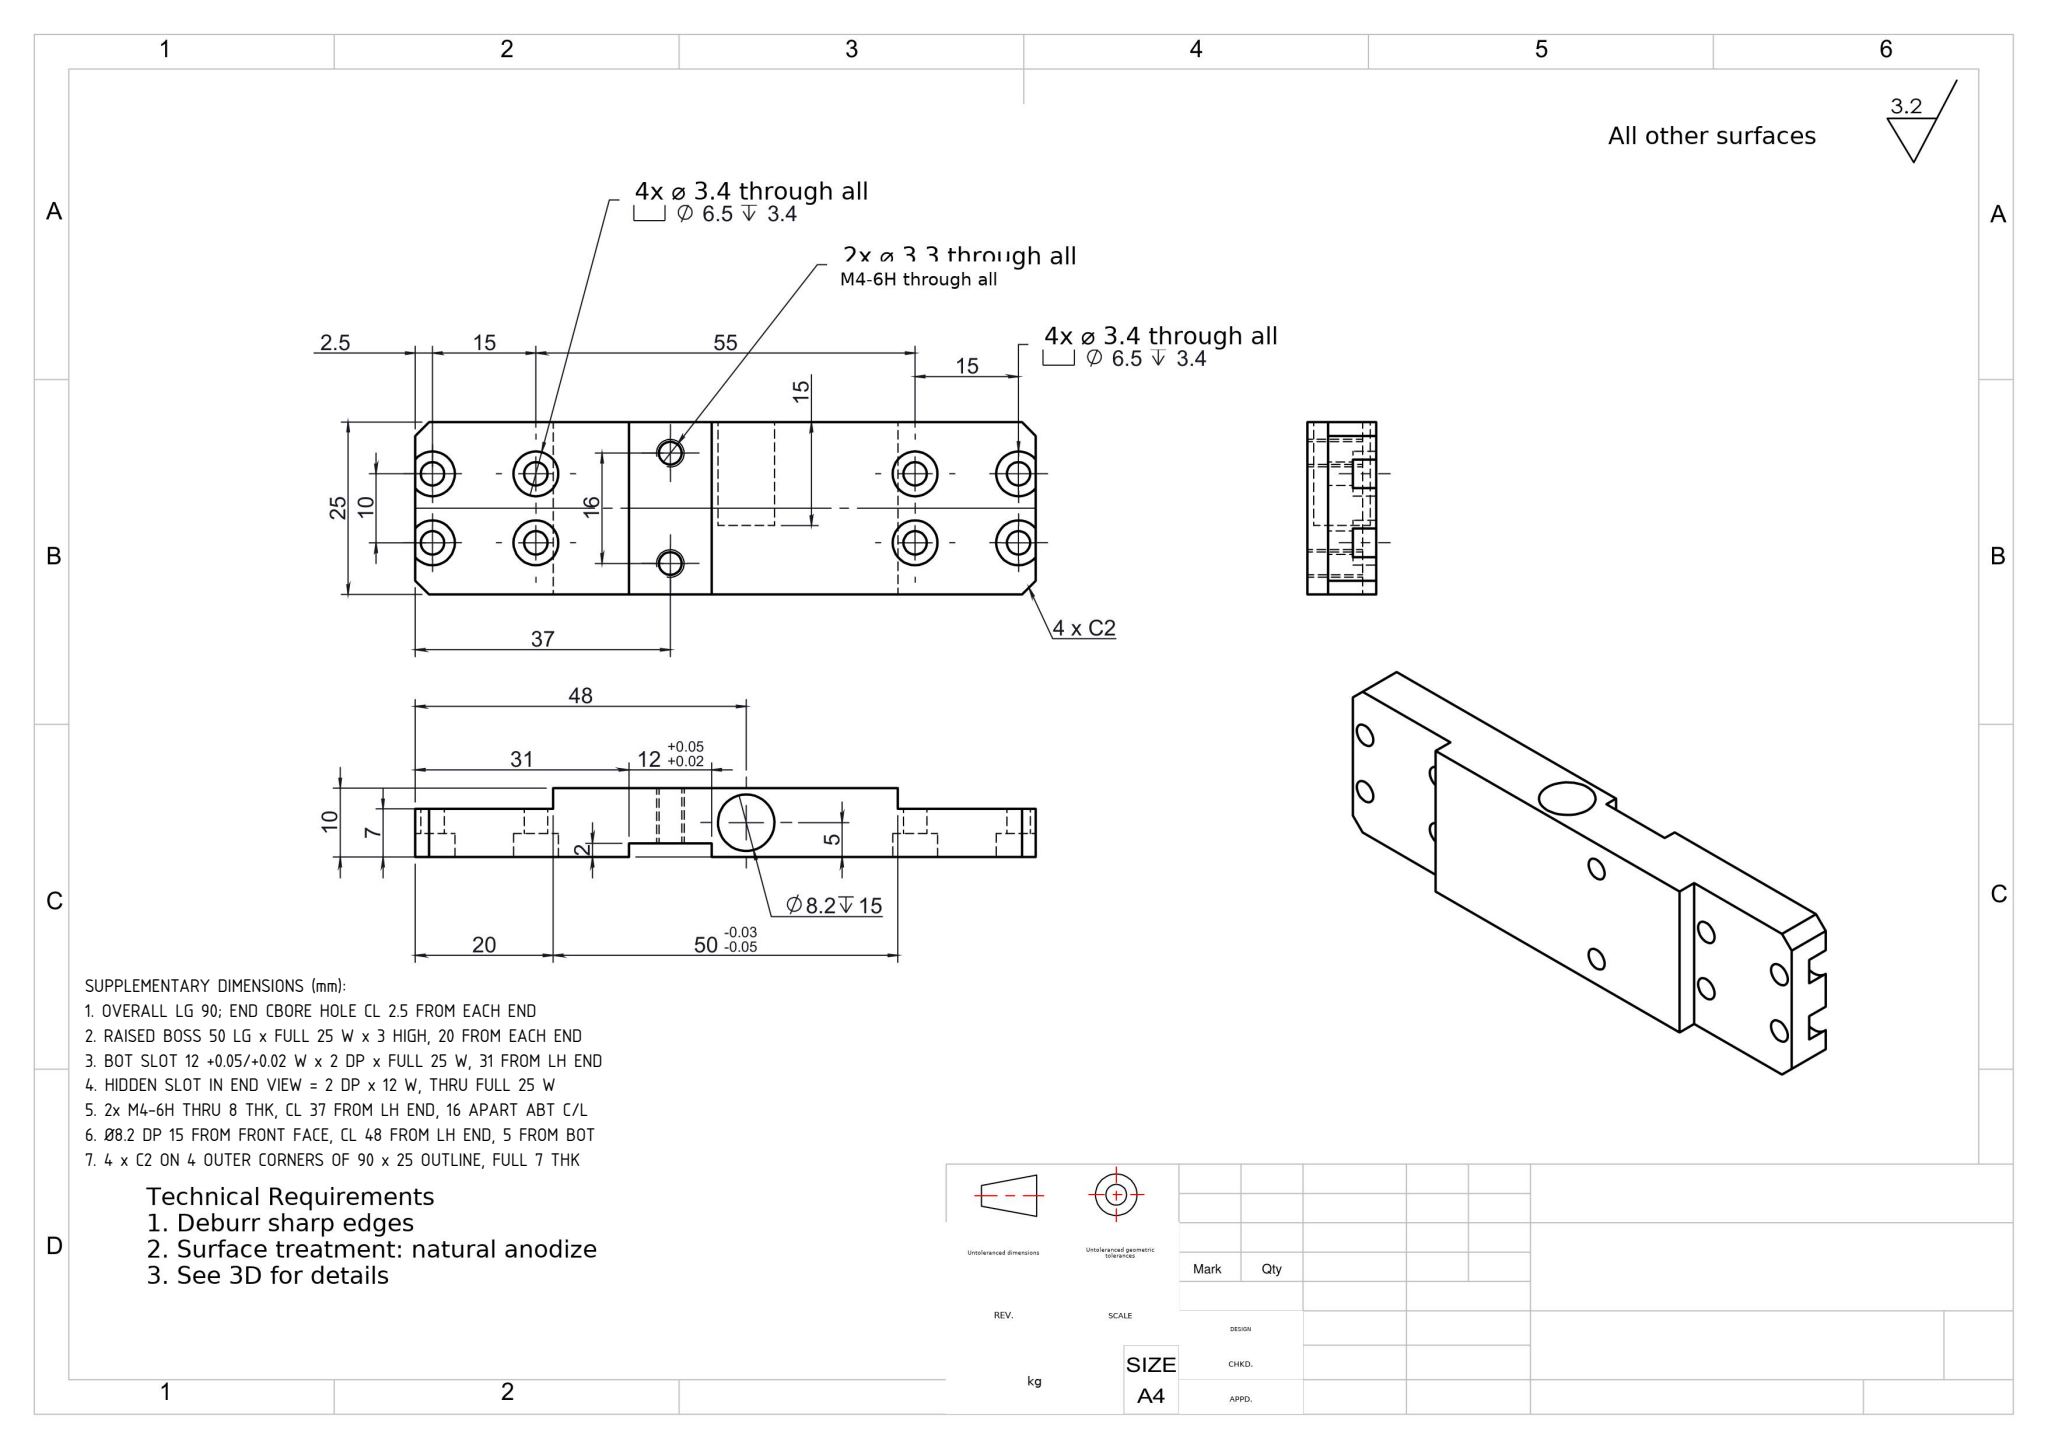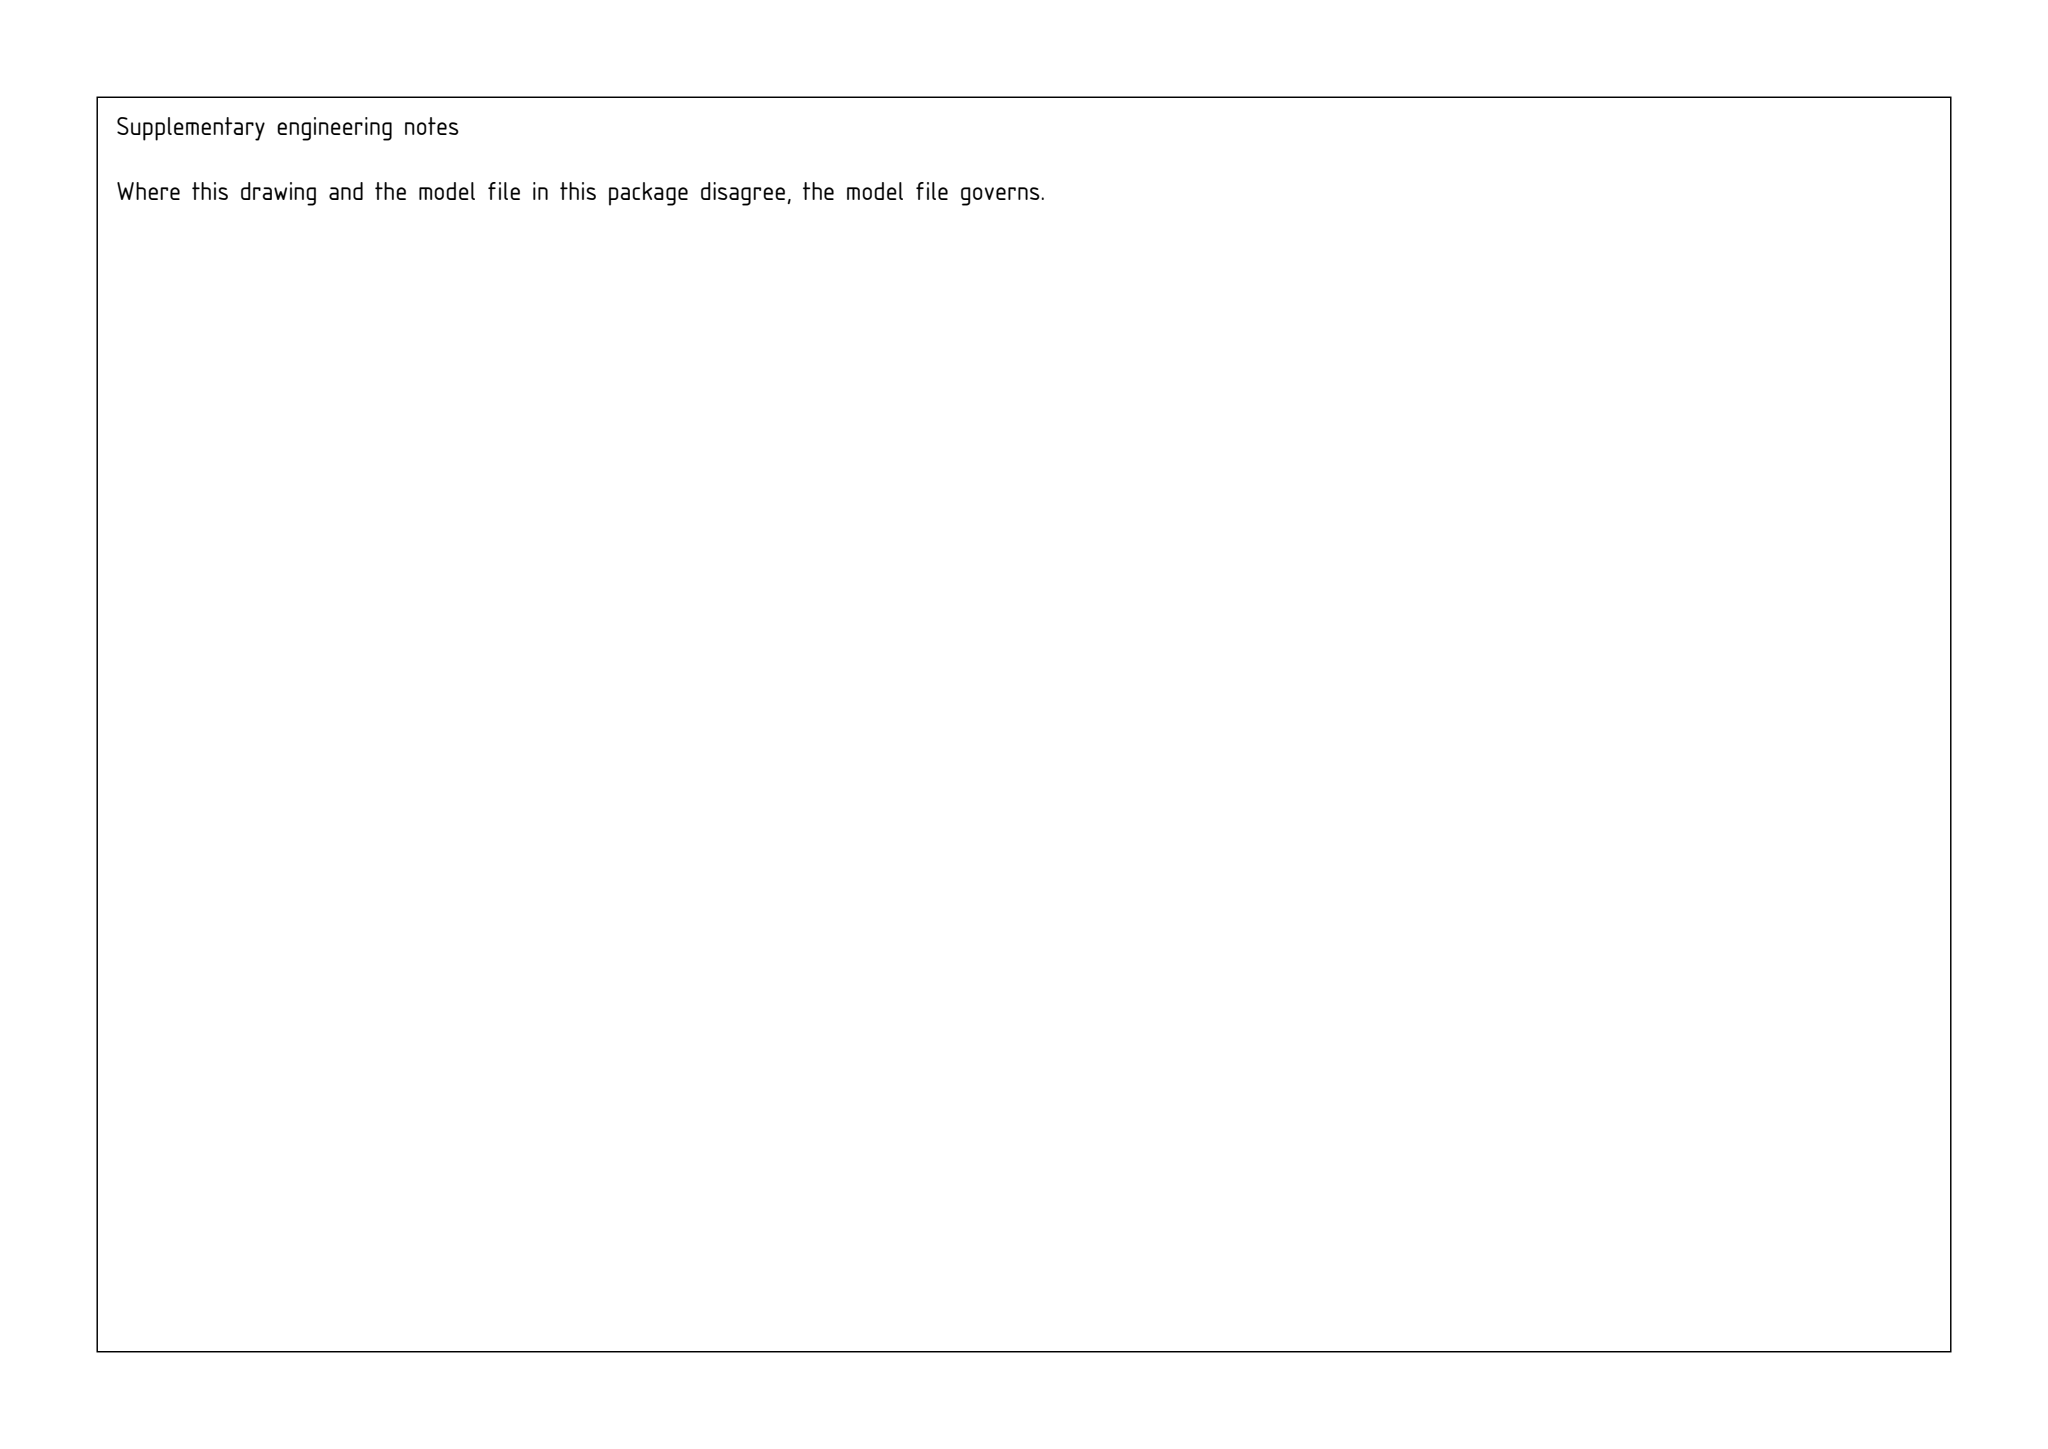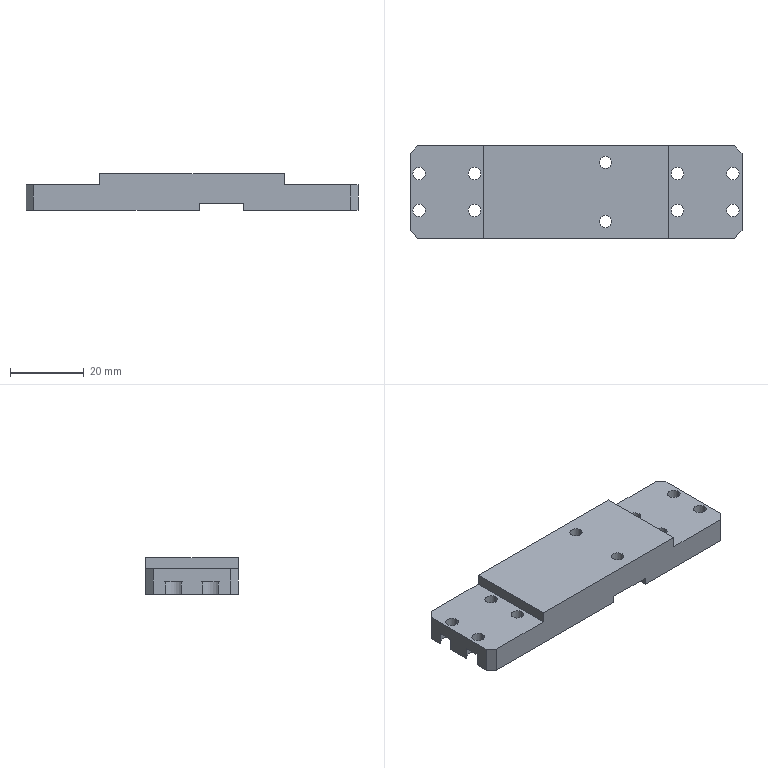Part | SolidWorks | mm | 1 solid | 63 faces | box 90 x 25 x 10 mm | volume 16780 mm3 | cylinder 36 | plane 27 | commonest cylinder face diameters 3.4 x16 6.5 x14 3.3 x4 8.2 x2
build123d program:
from build123d import *

# Parameters (mm, degrees)
SKETCH1_W                                       = 90
SKETCH1_H                                       = 25
BOSS_EXTRUDE1_DEPTH                             = 10
SKETCH2_W                                       = 20
SKETCH2_H                                       = 25
CUT_EXTRUDE1_DEPTH                              = 3
SKETCH3_W                                       = 12
SKETCH3_H                                       = 25
CUT_EXTRUDE2_DEPTH                              = 2
M3_HEX_SOCKET_HEAD_CAP_SCREW_CBORE1_D           = 3.4
M3_HEX_SOCKET_HEAD_CAP_SCREW_CBORE1_CBORE_D     = 6.5
M3_HEX_SOCKET_HEAD_CAP_SCREW_CBORE1_CBORE_DEPTH = 3.4
M3_HEX_SOCKET_HEAD_CAP_SCREW_CBORE2_D           = 3.4
M3_HEX_SOCKET_HEAD_CAP_SCREW_CBORE2_CBORE_D     = 6.5
M3_HEX_SOCKET_HEAD_CAP_SCREW_CBORE2_CBORE_DEPTH = 3.4
M4_TAPPED_HOLE1_D                               = 3.3
SKETCH10_R                                      = 4.1
CUT_EXTRUDE3_DEPTH                              = 15
CHAMFER1_SIZE                                   = 2


with BuildPart() as part:
    # Sketch1 → Boss-Extrude1 (new body)
    with BuildSketch(Plane.XY):
        Rectangle(SKETCH1_W, SKETCH1_H)
    extrude(amount=BOSS_EXTRUDE1_DEPTH)

    # Sketch2 → Cut-Extrude1 (cut)
    with BuildSketch(Plane.XY.offset(10)):
        with Locations((-35, 0)):
            Rectangle(SKETCH2_W, SKETCH2_H)
        with Locations((35, 0)):
            Rectangle(SKETCH2_W, SKETCH2_H)
    extrude(amount=-CUT_EXTRUDE1_DEPTH, mode=Mode.SUBTRACT)

    # Sketch3 → Cut-Extrude2 (cut)
    with BuildSketch(Plane(origin=(0, 0, 0), x_dir=(-1, 0, 0), z_dir=(0, 0, -1))):
        with Locations((-8, 0)):
            Rectangle(SKETCH3_W, SKETCH3_H)
    extrude(amount=-CUT_EXTRUDE2_DEPTH, mode=Mode.SUBTRACT)

    # M3 Hex Socket Head Cap Screw CBORE1 (through all)
    with Locations(Plane(origin=(0, 0, 0), x_dir=(-1, 0, 0), z_dir=(0, 0, -1))):
        with Locations((27.5, 5), (27.5, -5), (42.5, -5), (42.5, 5)):
            CounterBoreHole(M3_HEX_SOCKET_HEAD_CAP_SCREW_CBORE1_D / 2, M3_HEX_SOCKET_HEAD_CAP_SCREW_CBORE1_CBORE_D / 2, M3_HEX_SOCKET_HEAD_CAP_SCREW_CBORE1_CBORE_DEPTH)

    # M3 Hex Socket Head Cap Screw CBORE2 (through all)
    with Locations(Plane(origin=(0, 0, 0), x_dir=(-1, 0, 0), z_dir=(0, 0, -1))):
        with Locations((-42.5, 5), (-42.5, -5), (-27.5, 5), (-27.5, -5)):
            CounterBoreHole(M3_HEX_SOCKET_HEAD_CAP_SCREW_CBORE2_D / 2, M3_HEX_SOCKET_HEAD_CAP_SCREW_CBORE2_CBORE_D / 2, M3_HEX_SOCKET_HEAD_CAP_SCREW_CBORE2_CBORE_DEPTH)

    # M4 Tapped Hole1 (through all)
    with Locations(Plane(origin=(0, 0, 2), x_dir=(-1, 0, 0), z_dir=(0, 0, -1))):
        with Locations((-8, 8), (-8, -8)):
            Hole(M4_TAPPED_HOLE1_D / 2)

    # Sketch10 → Cut-Extrude3 (cut)
    with BuildSketch(Plane(origin=(0, 12.5, 0), x_dir=(1, 0, 0), z_dir=(0, 1, 0))):
        with Locations(Location((-3, -5, 0), (0, 0, 270))):
            Circle(SKETCH10_R)
    extrude(amount=-CUT_EXTRUDE3_DEPTH, mode=Mode.SUBTRACT)

    # Chamfer1
    chamfer1_edges = [part.edges().sort_by_distance(p)[0] for p in [
        (45, -12.5, 3.5),
        (-45, -12.5, 3.5),
        (-45, 12.5, 3.5),
        (45, 12.5, 3.5),
    ]]
    chamfer(chamfer1_edges, length=CHAMFER1_SIZE)


solid = part.part